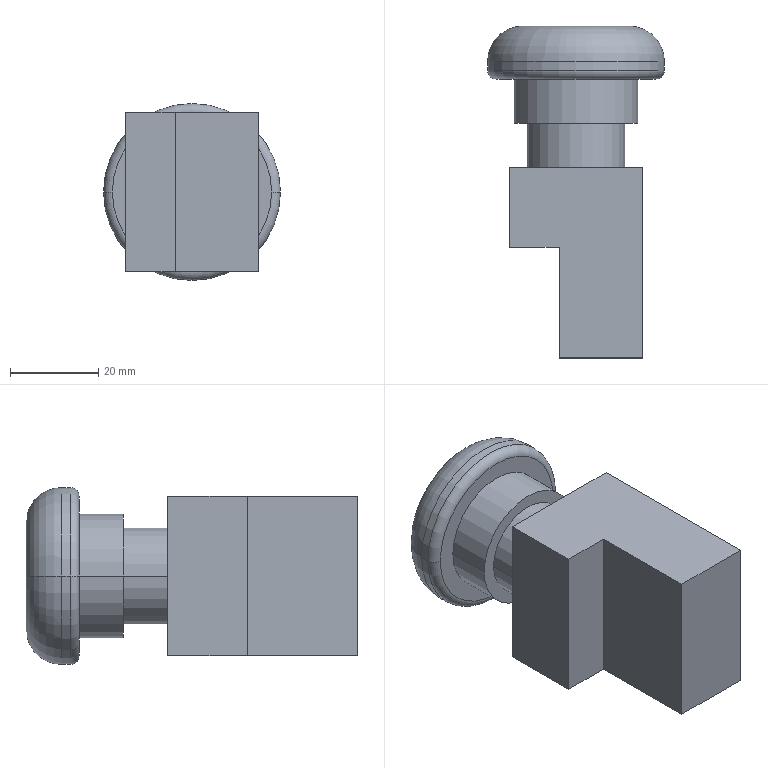Component | SolidWorks | EmergencyStopSwitch122-1 | 1 solid | 21 faces | box 40 x 75 x 40 mm | volume 59732 mm3 | plane 11 | cylinder 6 | torus 4 | commonest cylinder face diameters 22 x2 28 x2 40 x2
build123d program:
from build123d import *

# Parameters (mm, degrees)
EXTRUDE1_DEPTH      = 18
EXTRUDE1_DEPTH_BACK = 18
FILLET1_R           = 8
FILLET2_R           = 2


with BuildPart() as part:
    # Sketch1 → Extrude1 (new, two sides: drawn at the far end of the back side and taken through both)
    with BuildSketch(Plane.XY.offset(-EXTRUDE1_DEPTH_BACK)):
        Polygon((0, 0), (30, 0), (30, 18), (18.812, 18), (18.812, 43), (0, 43), align=None)
    extrude(amount=EXTRUDE1_DEPTH + EXTRUDE1_DEPTH_BACK)

    # Sketch2 → Revolve1 (revolve)
    with BuildSketch(Plane.XY, mode=Mode.PRIVATE) as revolve1_sk:
        Polygon((26, 0), (26, -10), (29, -10), (29, -20), (35, -20), (35, -32), (15, -32), (15, 0), align=None)
    revolve(revolve1_sk.sketch.rotate(Axis((15, 0, 0), (0, -1, 0)), 180), axis=Axis((15, 0, 0), (0, -1, 0)))

    # Fillet1
    fillet1_edges = [part.edges().sort_by_distance(p)[0] for p in [
        (35, -32, 0),
    ]]
    fillet(fillet1_edges, radius=FILLET1_R)

    # Fillet2
    fillet2_edges = [part.edges().sort_by_distance(p)[0] for p in [
        (35, -20, 0),
    ]]
    fillet(fillet2_edges, radius=FILLET2_R)


solid = part.part

# Placed as in the assembly
solid = solid.moved(Location((-497.479, 564.741, 730), (0, 0, 180)))
STEP:
#1=COLOUR_RGB('',0.7922,0.8196,0.9333);
#2=FILL_AREA_STYLE_COLOUR('',#1);
#3=FILL_AREA_STYLE('',(#2));
#4=SURFACE_STYLE_FILL_AREA(#3);
#5=SURFACE_SIDE_STYLE('',(#4));
#6=SURFACE_STYLE_USAGE(.BOTH.,#5);
#7=PRESENTATION_STYLE_ASSIGNMENT((#6));
#8=CARTESIAN_POINT('',(-19.468,23.021,28.74));
#9=VERTEX_POINT('',#8);
#10=CARTESIAN_POINT('',(-20.885,23.021,28.74));
#11=VERTEX_POINT('',#10);
#12=CARTESIAN_POINT('',(-20.176,23.021,28.74));
#13=DIRECTION('',(-0.,-1.,-0.));
#14=DIRECTION('',(-1.,0.,0.));
#15=AXIS2_PLACEMENT_3D('',#12,#13,#14);
#16=CIRCLE('',#15,0.7087);
#17=EDGE_CURVE('',#9,#11,#16,.T.);
#18=ORIENTED_EDGE('',*,*,#17,.F.);
#19=CARTESIAN_POINT('',(-19.389,23.1,28.74));
#20=VERTEX_POINT('',#19);
#21=CARTESIAN_POINT('',(-19.468,23.1,28.74));
#22=DIRECTION('',(-0.,0.,1.));
#23=DIRECTION('',(1.,0.,0.));
#24=AXIS2_PLACEMENT_3D('',#21,#22,#23);
#25=CIRCLE('',#24,0.07874);
#26=EDGE_CURVE('',#9,#20,#25,.T.);
#27=ORIENTED_EDGE('',*,*,#26,.T.);
#28=CARTESIAN_POINT('',(-20.964,23.1,28.74));
#29=VERTEX_POINT('',#28);
#30=CARTESIAN_POINT('',(-20.176,23.1,28.74));
#31=DIRECTION('',(0.,1.,0.));
#32=DIRECTION('',(-1.,0.,0.));
#33=AXIS2_PLACEMENT_3D('',#30,#31,#32);
#34=CIRCLE('',#33,0.7874);
#35=EDGE_CURVE('',#29,#20,#34,.T.);
#36=ORIENTED_EDGE('',*,*,#35,.F.);
#37=CARTESIAN_POINT('',(-20.885,23.1,28.74));
#38=DIRECTION('',(0.,0.,-1.));
#39=DIRECTION('',(0.,1.,0.));
#40=AXIS2_PLACEMENT_3D('',#37,#38,#39);
#41=CIRCLE('',#40,0.07874);
#42=EDGE_CURVE('',#11,#29,#41,.T.);
#43=ORIENTED_EDGE('',*,*,#42,.F.);
#44=EDGE_LOOP('',(#18,#27,#36,#43));
#45=FACE_OUTER_BOUND('',#44,.T.);
#46=CARTESIAN_POINT('',(-20.176,23.1,28.74));
#47=DIRECTION('',(0.,1.,0.));
#48=DIRECTION('',(-1.,0.,0.));
#49=AXIS2_PLACEMENT_3D('',#46,#47,#48);
#50=TOROIDAL_SURFACE('',#49,0.7087,0.07874);
#51=ADVANCED_FACE('',(#45),#50,.T.);
#52=CARTESIAN_POINT('',(-20.649,23.494,28.74));
#53=VERTEX_POINT('',#52);
#54=CARTESIAN_POINT('',(-19.704,23.494,28.74));
#55=VERTEX_POINT('',#54);
#56=CARTESIAN_POINT('',(-20.176,23.494,28.74));
#57=DIRECTION('',(0.,1.,0.));
#58=DIRECTION('',(1.,0.,0.));
#59=AXIS2_PLACEMENT_3D('',#56,#57,#58);
#60=CIRCLE('',#59,0.4724);
#61=EDGE_CURVE('',#53,#55,#60,.T.);
#62=ORIENTED_EDGE('',*,*,#61,.F.);
#63=CARTESIAN_POINT('',(-20.964,23.179,28.74));
#64=VERTEX_POINT('',#63);
#65=CARTESIAN_POINT('',(-20.649,23.179,28.74));
#66=DIRECTION('',(0.,-0.,1.));
#67=DIRECTION('',(1.,0.,0.));
#68=AXIS2_PLACEMENT_3D('',#65,#66,#67);
#69=CIRCLE('',#68,0.315);
#70=EDGE_CURVE('',#53,#64,#69,.T.);
#71=ORIENTED_EDGE('',*,*,#70,.T.);
#72=CARTESIAN_POINT('',(-19.389,23.179,28.74));
#73=VERTEX_POINT('',#72);
#74=CARTESIAN_POINT('',(-20.176,23.179,28.74));
#75=DIRECTION('',(-0.,-1.,-0.));
#76=DIRECTION('',(1.,0.,0.));
#77=AXIS2_PLACEMENT_3D('',#74,#75,#76);
#78=CIRCLE('',#77,0.7874);
#79=EDGE_CURVE('',#73,#64,#78,.T.);
#80=ORIENTED_EDGE('',*,*,#79,.F.);
#81=CARTESIAN_POINT('',(-19.704,23.179,28.74));
#82=DIRECTION('',(0.,0.,-1.));
#83=DIRECTION('',(0.,1.,0.));
#84=AXIS2_PLACEMENT_3D('',#81,#82,#83);
#85=CIRCLE('',#84,0.315);
#86=EDGE_CURVE('',#55,#73,#85,.T.);
#87=ORIENTED_EDGE('',*,*,#86,.F.);
#88=EDGE_LOOP('',(#62,#71,#80,#87));
#89=FACE_OUTER_BOUND('',#88,.T.);
#90=CARTESIAN_POINT('',(-20.176,23.179,28.74));
#91=DIRECTION('',(-0.,-1.,-0.));
#92=DIRECTION('',(1.,-0.,-0.));
#93=AXIS2_PLACEMENT_3D('',#90,#91,#92);
#94=TOROIDAL_SURFACE('',#93,0.4724,0.315);
#95=ADVANCED_FACE('',(#89),#94,.T.);
#96=CARTESIAN_POINT('',(-19.743,22.628,28.74));
#97=VERTEX_POINT('',#96);
#98=CARTESIAN_POINT('',(-20.609,22.628,28.74));
#99=VERTEX_POINT('',#98);
#100=CARTESIAN_POINT('',(-20.176,22.628,28.74));
#101=DIRECTION('',(-0.,-1.,-0.));
#102=DIRECTION('',(1.,0.,0.));
#103=AXIS2_PLACEMENT_3D('',#100,#101,#102);
#104=CIRCLE('',#103,0.4331);
#105=EDGE_CURVE('',#97,#99,#104,.T.);
#106=ORIENTED_EDGE('',*,*,#105,.T.);
#107=CARTESIAN_POINT('',(-20.609,22.234,28.74));
#108=VERTEX_POINT('',#107);
#109=CARTESIAN_POINT('',(-20.609,22.234,28.74));
#110=DIRECTION('',(-0.,-1.,-0.));
#111=VECTOR('',#110,39.37);
#112=LINE('',#109,#111);
#113=EDGE_CURVE('',#99,#108,#112,.T.);
#114=ORIENTED_EDGE('',*,*,#113,.T.);
#115=CARTESIAN_POINT('',(-19.743,22.234,28.74));
#116=VERTEX_POINT('',#115);
#117=CARTESIAN_POINT('',(-20.176,22.234,28.74));
#118=DIRECTION('',(0.,1.,0.));
#119=DIRECTION('',(0.,0.,1.));
#120=AXIS2_PLACEMENT_3D('',#117,#118,#119);
#121=CIRCLE('',#120,0.4331);
#122=EDGE_CURVE('',#108,#116,#121,.T.);
#123=ORIENTED_EDGE('',*,*,#122,.T.);
#124=CARTESIAN_POINT('',(-19.743,22.234,28.74));
#125=DIRECTION('',(-0.,-1.,-0.));
#126=VECTOR('',#125,39.37);
#127=LINE('',#124,#126);
#128=EDGE_CURVE('',#97,#116,#127,.T.);
#129=ORIENTED_EDGE('',*,*,#128,.F.);
#130=EDGE_LOOP('',(#106,#114,#123,#129));
#131=FACE_OUTER_BOUND('',#130,.T.);
#132=CARTESIAN_POINT('',(-20.176,22.234,28.74));
#133=DIRECTION('',(-0.,-1.,-0.));
#134=DIRECTION('',(1.,0.,0.));
#135=AXIS2_PLACEMENT_3D('',#132,#133,#134);
#136=CYLINDRICAL_SURFACE('',#135,0.4331);
#137=ADVANCED_FACE('',(#131),#136,.T.);
#138=CARTESIAN_POINT('',(-19.625,23.021,28.74));
#139=VERTEX_POINT('',#138);
#140=CARTESIAN_POINT('',(-20.728,23.021,28.74));
#141=VERTEX_POINT('',#140);
#142=CARTESIAN_POINT('',(-20.176,23.021,28.74));
#143=DIRECTION('',(-0.,-1.,-0.));
#144=DIRECTION('',(1.,0.,0.));
#145=AXIS2_PLACEMENT_3D('',#142,#143,#144);
#146=CIRCLE('',#145,0.5512);
#147=EDGE_CURVE('',#139,#141,#146,.T.);
#148=ORIENTED_EDGE('',*,*,#147,.T.);
#149=CARTESIAN_POINT('',(-20.728,22.628,28.74));
#150=VERTEX_POINT('',#149);
#151=CARTESIAN_POINT('',(-20.728,22.234,28.74));
#152=DIRECTION('',(-0.,-1.,-0.));
#153=VECTOR('',#152,39.37);
#154=LINE('',#151,#153);
#155=EDGE_CURVE('',#141,#150,#154,.T.);
#156=ORIENTED_EDGE('',*,*,#155,.T.);
#157=CARTESIAN_POINT('',(-19.625,22.628,28.74));
#158=VERTEX_POINT('',#157);
#159=CARTESIAN_POINT('',(-20.176,22.628,28.74));
#160=DIRECTION('',(-0.,-1.,-0.));
#161=DIRECTION('',(1.,0.,0.));
#162=AXIS2_PLACEMENT_3D('',#159,#160,#161);
#163=CIRCLE('',#162,0.5512);
#164=EDGE_CURVE('',#158,#150,#163,.T.);
#165=ORIENTED_EDGE('',*,*,#164,.F.);
#166=CARTESIAN_POINT('',(-19.625,22.234,28.74));
#167=DIRECTION('',(-0.,-1.,-0.));
#168=VECTOR('',#167,39.37);
#169=LINE('',#166,#168);
#170=EDGE_CURVE('',#139,#158,#169,.T.);
#171=ORIENTED_EDGE('',*,*,#170,.F.);
#172=EDGE_LOOP('',(#148,#156,#165,#171));
#173=FACE_OUTER_BOUND('',#172,.T.);
#174=CARTESIAN_POINT('',(-20.176,22.234,28.74));
#175=DIRECTION('',(-0.,-1.,-0.));
#176=DIRECTION('',(1.,0.,0.));
#177=AXIS2_PLACEMENT_3D('',#174,#175,#176);
#178=CYLINDRICAL_SURFACE('',#177,0.5512);
#179=ADVANCED_FACE('',(#173),#178,.T.);
#180=ORIENTED_EDGE('',*,*,#79,.T.);
#181=CARTESIAN_POINT('',(-20.964,22.234,28.74));
#182=DIRECTION('',(-0.,-1.,-0.));
#183=VECTOR('',#182,39.37);
#184=LINE('',#181,#183);
#185=EDGE_CURVE('',#64,#29,#184,.T.);
#186=ORIENTED_EDGE('',*,*,#185,.T.);
#187=ORIENTED_EDGE('',*,*,#35,.T.);
#188=CARTESIAN_POINT('',(-19.389,22.234,28.74));
#189=DIRECTION('',(-0.,-1.,-0.));
#190=VECTOR('',#189,39.37);
#191=LINE('',#188,#190);
#192=EDGE_CURVE('',#73,#20,#191,.T.);
#193=ORIENTED_EDGE('',*,*,#192,.F.);
#194=EDGE_LOOP('',(#180,#186,#187,#193));
#195=FACE_OUTER_BOUND('',#194,.T.);
#196=CARTESIAN_POINT('',(-20.176,22.234,28.74));
#197=DIRECTION('',(-0.,-1.,-0.));
#198=DIRECTION('',(1.,0.,0.));
#199=AXIS2_PLACEMENT_3D('',#196,#197,#198);
#200=CYLINDRICAL_SURFACE('',#199,0.7874);
#201=ADVANCED_FACE('',(#195),#200,.T.);
#202=CARTESIAN_POINT('',(-19.586,22.234,29.449));
#203=VERTEX_POINT('',#202);
#204=CARTESIAN_POINT('',(-19.586,22.234,28.031));
#205=VERTEX_POINT('',#204);
#206=CARTESIAN_POINT('',(-19.586,22.234,29.449));
#207=DIRECTION('',(0.,0.,-1.));
#208=VECTOR('',#207,39.37);
#209=LINE('',#206,#208);
#210=EDGE_CURVE('',#203,#205,#209,.T.);
#211=ORIENTED_EDGE('',*,*,#210,.T.);
#212=CARTESIAN_POINT('',(-20.767,22.234,28.031));
#213=VERTEX_POINT('',#212);
#214=CARTESIAN_POINT('',(-19.586,22.234,28.031));
#215=DIRECTION('',(-1.,0.,0.));
#216=VECTOR('',#215,39.37);
#217=LINE('',#214,#216);
#218=EDGE_CURVE('',#205,#213,#217,.T.);
#219=ORIENTED_EDGE('',*,*,#218,.T.);
#220=CARTESIAN_POINT('',(-20.767,22.234,29.449));
#221=VERTEX_POINT('',#220);
#222=CARTESIAN_POINT('',(-20.767,22.234,29.449));
#223=DIRECTION('',(0.,0.,-1.));
#224=VECTOR('',#223,39.37);
#225=LINE('',#222,#224);
#226=EDGE_CURVE('',#221,#213,#225,.T.);
#227=ORIENTED_EDGE('',*,*,#226,.F.);
#228=CARTESIAN_POINT('',(-19.586,22.234,29.449));
#229=DIRECTION('',(-1.,0.,0.));
#230=VECTOR('',#229,39.37);
#231=LINE('',#228,#230);
#232=EDGE_CURVE('',#203,#221,#231,.T.);
#233=ORIENTED_EDGE('',*,*,#232,.F.);
#234=EDGE_LOOP('',(#211,#219,#227,#233));
#235=FACE_OUTER_BOUND('',#234,.T.);
#236=CARTESIAN_POINT('',(-20.176,22.234,28.74));
#237=DIRECTION('',(0.,1.,0.));
#238=DIRECTION('',(0.,0.,1.));
#239=AXIS2_PLACEMENT_3D('',#236,#237,#238);
#240=CIRCLE('',#239,0.4331);
#241=EDGE_CURVE('',#116,#108,#240,.T.);
#242=ORIENTED_EDGE('',*,*,#241,.F.);
#243=ORIENTED_EDGE('',*,*,#122,.F.);
#244=EDGE_LOOP('',(#242,#243));
#245=FACE_BOUND('',#244,.T.);
#246=CARTESIAN_POINT('',(-19.586,22.234,29.449));
#247=DIRECTION('',(-0.,-1.,-0.));
#248=DIRECTION('',(-0.,-0.,1.));
#249=AXIS2_PLACEMENT_3D('',#246,#247,#248);
#250=PLANE('',#249);
#251=ADVANCED_FACE('',(#235,#245),#250,.F.);
#252=CARTESIAN_POINT('',(-19.586,20.541,29.449));
#253=VERTEX_POINT('',#252);
#254=CARTESIAN_POINT('',(-19.586,20.541,28.031));
#255=VERTEX_POINT('',#254);
#256=CARTESIAN_POINT('',(-19.586,20.541,29.449));
#257=DIRECTION('',(0.,0.,-1.));
#258=VECTOR('',#257,39.37);
#259=LINE('',#256,#258);
#260=EDGE_CURVE('',#253,#255,#259,.T.);
#261=ORIENTED_EDGE('',*,*,#260,.T.);
#262=CARTESIAN_POINT('',(-19.586,22.234,28.031));
#263=DIRECTION('',(0.,1.,0.));
#264=VECTOR('',#263,39.37);
#265=LINE('',#262,#264);
#266=EDGE_CURVE('',#255,#205,#265,.T.);
#267=ORIENTED_EDGE('',*,*,#266,.T.);
#268=ORIENTED_EDGE('',*,*,#210,.F.);
#269=CARTESIAN_POINT('',(-19.586,22.234,29.449));
#270=DIRECTION('',(0.,1.,0.));
#271=VECTOR('',#270,39.37);
#272=LINE('',#269,#271);
#273=EDGE_CURVE('',#253,#203,#272,.T.);
#274=ORIENTED_EDGE('',*,*,#273,.F.);
#275=EDGE_LOOP('',(#261,#267,#268,#274));
#276=FACE_OUTER_BOUND('',#275,.T.);
#277=CARTESIAN_POINT('',(-19.586,22.234,29.449));
#278=DIRECTION('',(-1.,0.,0.));
#279=DIRECTION('',(0.,0.,-1.));
#280=AXIS2_PLACEMENT_3D('',#277,#278,#279);
#281=PLANE('',#280);
#282=ADVANCED_FACE('',(#276),#281,.F.);
#283=ORIENTED_EDGE('',*,*,#226,.T.);
#284=CARTESIAN_POINT('',(-20.767,21.525,28.031));
#285=VERTEX_POINT('',#284);
#286=CARTESIAN_POINT('',(-20.767,22.234,28.031));
#287=DIRECTION('',(-0.,-1.,-0.));
#288=VECTOR('',#287,39.37);
#289=LINE('',#286,#288);
#290=EDGE_CURVE('',#213,#285,#289,.T.);
#291=ORIENTED_EDGE('',*,*,#290,.T.);
#292=CARTESIAN_POINT('',(-20.767,21.525,29.449));
#293=VERTEX_POINT('',#292);
#294=CARTESIAN_POINT('',(-20.767,21.525,29.449));
#295=DIRECTION('',(0.,0.,-1.));
#296=VECTOR('',#295,39.37);
#297=LINE('',#294,#296);
#298=EDGE_CURVE('',#293,#285,#297,.T.);
#299=ORIENTED_EDGE('',*,*,#298,.F.);
#300=CARTESIAN_POINT('',(-20.767,22.234,29.449));
#301=DIRECTION('',(-0.,-1.,-0.));
#302=VECTOR('',#301,39.37);
#303=LINE('',#300,#302);
#304=EDGE_CURVE('',#221,#293,#303,.T.);
#305=ORIENTED_EDGE('',*,*,#304,.F.);
#306=EDGE_LOOP('',(#283,#291,#299,#305));
#307=FACE_OUTER_BOUND('',#306,.T.);
#308=CARTESIAN_POINT('',(-20.767,22.234,29.449));
#309=DIRECTION('',(1.,-0.,0.));
#310=DIRECTION('',(-0.,-0.,1.));
#311=AXIS2_PLACEMENT_3D('',#308,#309,#310);
#312=PLANE('',#311);
#313=ADVANCED_FACE('',(#307),#312,.F.);
#314=ORIENTED_EDGE('',*,*,#298,.T.);
#315=CARTESIAN_POINT('',(-20.326,21.525,28.031));
#316=VERTEX_POINT('',#315);
#317=CARTESIAN_POINT('',(-20.767,21.525,28.031));
#318=DIRECTION('',(1.,-0.,0.));
#319=VECTOR('',#318,39.37);
#320=LINE('',#317,#319);
#321=EDGE_CURVE('',#285,#316,#320,.T.);
#322=ORIENTED_EDGE('',*,*,#321,.T.);
#323=CARTESIAN_POINT('',(-20.326,21.525,29.449));
#324=VERTEX_POINT('',#323);
#325=CARTESIAN_POINT('',(-20.326,21.525,29.449));
#326=DIRECTION('',(0.,0.,-1.));
#327=VECTOR('',#326,39.37);
#328=LINE('',#325,#327);
#329=EDGE_CURVE('',#324,#316,#328,.T.);
#330=ORIENTED_EDGE('',*,*,#329,.F.);
#331=CARTESIAN_POINT('',(-20.767,21.525,29.449));
#332=DIRECTION('',(1.,-0.,0.));
#333=VECTOR('',#332,39.37);
#334=LINE('',#331,#333);
#335=EDGE_CURVE('',#293,#324,#334,.T.);
#336=ORIENTED_EDGE('',*,*,#335,.F.);
#337=EDGE_LOOP('',(#314,#322,#330,#336));
#338=FACE_OUTER_BOUND('',#337,.T.);
#339=CARTESIAN_POINT('',(-20.767,21.525,29.449));
#340=DIRECTION('',(0.,1.,0.));
#341=DIRECTION('',(0.,0.,-1.));
#342=AXIS2_PLACEMENT_3D('',#339,#340,#341);
#343=PLANE('',#342);
#344=ADVANCED_FACE('',(#338),#343,.F.);
#345=ORIENTED_EDGE('',*,*,#329,.T.);
#346=CARTESIAN_POINT('',(-20.326,20.541,28.031));
#347=VERTEX_POINT('',#346);
#348=CARTESIAN_POINT('',(-20.326,20.541,28.031));
#349=DIRECTION('',(0.,-1.,-0.));
#350=VECTOR('',#349,39.37);
#351=LINE('',#348,#350);
#352=EDGE_CURVE('',#316,#347,#351,.T.);
#353=ORIENTED_EDGE('',*,*,#352,.T.);
#354=CARTESIAN_POINT('',(-20.326,20.541,29.449));
#355=VERTEX_POINT('',#354);
#356=CARTESIAN_POINT('',(-20.326,20.541,29.449));
#357=DIRECTION('',(0.,0.,-1.));
#358=VECTOR('',#357,39.37);
#359=LINE('',#356,#358);
#360=EDGE_CURVE('',#355,#347,#359,.T.);
#361=ORIENTED_EDGE('',*,*,#360,.F.);
#362=CARTESIAN_POINT('',(-20.326,20.541,29.449));
#363=DIRECTION('',(0.,-1.,-0.));
#364=VECTOR('',#363,39.37);
#365=LINE('',#362,#364);
#366=EDGE_CURVE('',#324,#355,#365,.T.);
#367=ORIENTED_EDGE('',*,*,#366,.F.);
#368=EDGE_LOOP('',(#345,#353,#361,#367));
#369=FACE_OUTER_BOUND('',#368,.T.);
#370=CARTESIAN_POINT('',(-20.326,20.541,29.449));
#371=DIRECTION('',(1.,0.,0.));
#372=DIRECTION('',(-0.,1.,0.));
#373=AXIS2_PLACEMENT_3D('',#370,#371,#372);
#374=PLANE('',#373);
#375=ADVANCED_FACE('',(#369),#374,.F.);
#376=ORIENTED_EDGE('',*,*,#360,.T.);
#377=CARTESIAN_POINT('',(-19.586,20.541,28.031));
#378=DIRECTION('',(1.,-0.,0.));
#379=VECTOR('',#378,39.37);
#380=LINE('',#377,#379);
#381=EDGE_CURVE('',#347,#255,#380,.T.);
#382=ORIENTED_EDGE('',*,*,#381,.T.);
#383=ORIENTED_EDGE('',*,*,#260,.F.);
#384=CARTESIAN_POINT('',(-19.586,20.541,29.449));
#385=DIRECTION('',(1.,-0.,0.));
#386=VECTOR('',#385,39.37);
#387=LINE('',#384,#386);
#388=EDGE_CURVE('',#355,#253,#387,.T.);
#389=ORIENTED_EDGE('',*,*,#388,.F.);
#390=EDGE_LOOP('',(#376,#382,#383,#389));
#391=FACE_OUTER_BOUND('',#390,.T.);
#392=CARTESIAN_POINT('',(-19.586,20.541,29.449));
#393=DIRECTION('',(0.,1.,0.));
#394=DIRECTION('',(0.,0.,-1.));
#395=AXIS2_PLACEMENT_3D('',#392,#393,#394);
#396=PLANE('',#395);
#397=ADVANCED_FACE('',(#391),#396,.F.);
#398=ORIENTED_EDGE('',*,*,#273,.T.);
#399=ORIENTED_EDGE('',*,*,#232,.T.);
#400=ORIENTED_EDGE('',*,*,#304,.T.);
#401=ORIENTED_EDGE('',*,*,#335,.T.);
#402=ORIENTED_EDGE('',*,*,#366,.T.);
#403=ORIENTED_EDGE('',*,*,#388,.T.);
#404=EDGE_LOOP('',(#398,#399,#400,#401,#402,#403));
#405=FACE_OUTER_BOUND('',#404,.T.);
#406=CARTESIAN_POINT('',(-19.586,20.541,29.449));
#407=DIRECTION('',(0.,0.,-1.));
#408=DIRECTION('',(1.,-0.,0.));
#409=AXIS2_PLACEMENT_3D('',#406,#407,#408);
#410=PLANE('',#409);
#411=ADVANCED_FACE('',(#405),#410,.F.);
#412=ORIENTED_EDGE('',*,*,#266,.F.);
#413=ORIENTED_EDGE('',*,*,#381,.F.);
#414=ORIENTED_EDGE('',*,*,#352,.F.);
#415=ORIENTED_EDGE('',*,*,#321,.F.);
#416=ORIENTED_EDGE('',*,*,#290,.F.);
#417=ORIENTED_EDGE('',*,*,#218,.F.);
#418=EDGE_LOOP('',(#412,#413,#414,#415,#416,#417));
#419=FACE_OUTER_BOUND('',#418,.T.);
#420=CARTESIAN_POINT('',(-19.586,20.541,28.031));
#421=DIRECTION('',(0.,0.,-1.));
#422=DIRECTION('',(1.,-0.,0.));
#423=AXIS2_PLACEMENT_3D('',#420,#421,#422);
#424=PLANE('',#423);
#425=ADVANCED_FACE('',(#419),#424,.T.);
#426=CARTESIAN_POINT('',(-20.176,23.494,28.74));
#427=DIRECTION('',(0.,1.,0.));
#428=DIRECTION('',(1.,0.,0.));
#429=AXIS2_PLACEMENT_3D('',#426,#427,#428);
#430=CIRCLE('',#429,0.4724);
#431=EDGE_CURVE('',#55,#53,#430,.T.);
#432=ORIENTED_EDGE('',*,*,#431,.T.);
#433=ORIENTED_EDGE('',*,*,#61,.T.);
#434=EDGE_LOOP('',(#432,#433));
#435=FACE_OUTER_BOUND('',#434,.T.);
#436=CARTESIAN_POINT('',(-20.176,23.494,28.74));
#437=DIRECTION('',(-0.,-1.,-0.));
#438=DIRECTION('',(1.,-0.,-0.));
#439=AXIS2_PLACEMENT_3D('',#436,#437,#438);
#440=PLANE('',#439);
#441=ADVANCED_FACE('',(#435),#440,.F.);
#442=ORIENTED_EDGE('',*,*,#185,.F.);
#443=CARTESIAN_POINT('',(-20.176,23.179,28.74));
#444=DIRECTION('',(-0.,-1.,-0.));
#445=DIRECTION('',(1.,0.,0.));
#446=AXIS2_PLACEMENT_3D('',#443,#444,#445);
#447=CIRCLE('',#446,0.7874);
#448=EDGE_CURVE('',#64,#73,#447,.T.);
#449=ORIENTED_EDGE('',*,*,#448,.T.);
#450=ORIENTED_EDGE('',*,*,#192,.T.);
#451=CARTESIAN_POINT('',(-20.176,23.1,28.74));
#452=DIRECTION('',(0.,1.,0.));
#453=DIRECTION('',(-1.,0.,0.));
#454=AXIS2_PLACEMENT_3D('',#451,#452,#453);
#455=CIRCLE('',#454,0.7874);
#456=EDGE_CURVE('',#20,#29,#455,.T.);
#457=ORIENTED_EDGE('',*,*,#456,.T.);
#458=EDGE_LOOP('',(#442,#449,#450,#457));
#459=FACE_OUTER_BOUND('',#458,.T.);
#460=CARTESIAN_POINT('',(-20.176,22.234,28.74));
#461=DIRECTION('',(-0.,-1.,-0.));
#462=DIRECTION('',(1.,0.,0.));
#463=AXIS2_PLACEMENT_3D('',#460,#461,#462);
#464=CYLINDRICAL_SURFACE('',#463,0.7874);
#465=ADVANCED_FACE('',(#459),#464,.T.);
#466=CARTESIAN_POINT('',(-20.176,23.021,28.74));
#467=DIRECTION('',(-0.,-1.,-0.));
#468=DIRECTION('',(-1.,0.,0.));
#469=AXIS2_PLACEMENT_3D('',#466,#467,#468);
#470=CIRCLE('',#469,0.7087);
#471=EDGE_CURVE('',#11,#9,#470,.T.);
#472=ORIENTED_EDGE('',*,*,#471,.T.);
#473=ORIENTED_EDGE('',*,*,#17,.T.);
#474=EDGE_LOOP('',(#472,#473));
#475=FACE_OUTER_BOUND('',#474,.T.);
#476=ORIENTED_EDGE('',*,*,#147,.F.);
#477=CARTESIAN_POINT('',(-20.176,23.021,28.74));
#478=DIRECTION('',(-0.,-1.,-0.));
#479=DIRECTION('',(1.,0.,0.));
#480=AXIS2_PLACEMENT_3D('',#477,#478,#479);
#481=CIRCLE('',#480,0.5512);
#482=EDGE_CURVE('',#141,#139,#481,.T.);
#483=ORIENTED_EDGE('',*,*,#482,.F.);
#484=EDGE_LOOP('',(#476,#483));
#485=FACE_BOUND('',#484,.T.);
#486=CARTESIAN_POINT('',(-20.728,23.021,28.74));
#487=DIRECTION('',(0.,1.,0.));
#488=DIRECTION('',(-1.,0.,0.));
#489=AXIS2_PLACEMENT_3D('',#486,#487,#488);
#490=PLANE('',#489);
#491=ADVANCED_FACE('',(#475,#485),#490,.F.);
#492=ORIENTED_EDGE('',*,*,#155,.F.);
#493=ORIENTED_EDGE('',*,*,#482,.T.);
#494=ORIENTED_EDGE('',*,*,#170,.T.);
#495=CARTESIAN_POINT('',(-20.176,22.628,28.74));
#496=DIRECTION('',(-0.,-1.,-0.));
#497=DIRECTION('',(1.,0.,0.));
#498=AXIS2_PLACEMENT_3D('',#495,#496,#497);
#499=CIRCLE('',#498,0.5512);
#500=EDGE_CURVE('',#150,#158,#499,.T.);
#501=ORIENTED_EDGE('',*,*,#500,.F.);
#502=EDGE_LOOP('',(#492,#493,#494,#501));
#503=FACE_OUTER_BOUND('',#502,.T.);
#504=CARTESIAN_POINT('',(-20.176,22.234,28.74));
#505=DIRECTION('',(-0.,-1.,-0.));
#506=DIRECTION('',(1.,0.,0.));
#507=AXIS2_PLACEMENT_3D('',#504,#505,#506);
#508=CYLINDRICAL_SURFACE('',#507,0.5512);
#509=ADVANCED_FACE('',(#503),#508,.T.);
#510=ORIENTED_EDGE('',*,*,#105,.F.);
#511=CARTESIAN_POINT('',(-20.176,22.628,28.74));
#512=DIRECTION('',(-0.,-1.,-0.));
#513=DIRECTION('',(1.,0.,0.));
#514=AXIS2_PLACEMENT_3D('',#511,#512,#513);
#515=CIRCLE('',#514,0.4331);
#516=EDGE_CURVE('',#99,#97,#515,.T.);
#517=ORIENTED_EDGE('',*,*,#516,.F.);
#518=EDGE_LOOP('',(#510,#517));
#519=FACE_BOUND('',#518,.T.);
#520=ORIENTED_EDGE('',*,*,#164,.T.);
#521=ORIENTED_EDGE('',*,*,#500,.T.);
#522=EDGE_LOOP('',(#520,#521));
#523=FACE_OUTER_BOUND('',#522,.T.);
#524=CARTESIAN_POINT('',(-20.609,22.628,28.74));
#525=DIRECTION('',(0.,1.,0.));
#526=DIRECTION('',(-1.,0.,0.));
#527=AXIS2_PLACEMENT_3D('',#524,#525,#526);
#528=PLANE('',#527);
#529=ADVANCED_FACE('',(#519,#523),#528,.F.);
#530=ORIENTED_EDGE('',*,*,#113,.F.);
#531=ORIENTED_EDGE('',*,*,#516,.T.);
#532=ORIENTED_EDGE('',*,*,#128,.T.);
#533=ORIENTED_EDGE('',*,*,#241,.T.);
#534=EDGE_LOOP('',(#530,#531,#532,#533));
#535=FACE_OUTER_BOUND('',#534,.T.);
#536=CARTESIAN_POINT('',(-20.176,22.234,28.74));
#537=DIRECTION('',(-0.,-1.,-0.));
#538=DIRECTION('',(1.,0.,0.));
#539=AXIS2_PLACEMENT_3D('',#536,#537,#538);
#540=CYLINDRICAL_SURFACE('',#539,0.4331);
#541=ADVANCED_FACE('',(#535),#540,.T.);
#542=ORIENTED_EDGE('',*,*,#70,.F.);
#543=ORIENTED_EDGE('',*,*,#431,.F.);
#544=ORIENTED_EDGE('',*,*,#86,.T.);
#545=ORIENTED_EDGE('',*,*,#448,.F.);
#546=EDGE_LOOP('',(#542,#543,#544,#545));
#547=FACE_OUTER_BOUND('',#546,.T.);
#548=CARTESIAN_POINT('',(-20.176,23.179,28.74));
#549=DIRECTION('',(-0.,-1.,-0.));
#550=DIRECTION('',(1.,-0.,-0.));
#551=AXIS2_PLACEMENT_3D('',#548,#549,#550);
#552=TOROIDAL_SURFACE('',#551,0.4724,0.315);
#553=ADVANCED_FACE('',(#547),#552,.T.);
#554=ORIENTED_EDGE('',*,*,#26,.F.);
#555=ORIENTED_EDGE('',*,*,#471,.F.);
#556=ORIENTED_EDGE('',*,*,#42,.T.);
#557=ORIENTED_EDGE('',*,*,#456,.F.);
#558=EDGE_LOOP('',(#554,#555,#556,#557));
#559=FACE_OUTER_BOUND('',#558,.T.);
#560=CARTESIAN_POINT('',(-20.176,23.1,28.74));
#561=DIRECTION('',(0.,1.,0.));
#562=DIRECTION('',(-1.,0.,0.));
#563=AXIS2_PLACEMENT_3D('',#560,#561,#562);
#564=TOROIDAL_SURFACE('',#563,0.7087,0.07874);
#565=ADVANCED_FACE('',(#559),#564,.T.);
#566=CLOSED_SHELL('',(#51,#95,#137,#179,#201,#251,#282,#313,#344,#375,#397,#411,#425,#441,#465,#491,#509,#529,#541,#553,#565));
#567=MANIFOLD_SOLID_BREP('',#566);
#568=STYLED_ITEM('',(#7),#567);
#569=(LENGTH_UNIT()NAMED_UNIT(*)SI_UNIT($,.METRE.));
#570=LENGTH_MEASURE_WITH_UNIT(LENGTH_MEASURE(0.0254),#569);
#571=DIMENSIONAL_EXPONENTS(1.,0.,0.,0.,0.,0.,0.);
#572=(CONVERSION_BASED_UNIT('',#570)LENGTH_UNIT()NAMED_UNIT(#571));
#573=UNCERTAINTY_MEASURE_WITH_UNIT(LENGTH_MEASURE(0.00001),#572,'','');
#574=(NAMED_UNIT(*)PLANE_ANGLE_UNIT()SI_UNIT($,.RADIAN.));
#575=(NAMED_UNIT(*)SI_UNIT($,.STERADIAN.)SOLID_ANGLE_UNIT());
#576=(GEOMETRIC_REPRESENTATION_CONTEXT(3)GLOBAL_UNCERTAINTY_ASSIGNED_CONTEXT((#573))GLOBAL_UNIT_ASSIGNED_CONTEXT((#572,#574,#575))REPRESENTATION_CONTEXT('',''));
#577=MECHANICAL_DESIGN_GEOMETRIC_PRESENTATION_REPRESENTATION('',(#568),#576);
#578=CARTESIAN_POINT('',(0.,0.,0.));
#579=DIRECTION('',(0.,0.,1.));
#580=DIRECTION('',(1.,0.,0.));
#581=AXIS2_PLACEMENT_3D('',#578,#579,#580);
#582=(LENGTH_UNIT()NAMED_UNIT(*)SI_UNIT($,.METRE.));
#583=LENGTH_MEASURE_WITH_UNIT(LENGTH_MEASURE(0.0254),#582);
#584=DIMENSIONAL_EXPONENTS(1.,0.,0.,0.,0.,0.,0.);
#585=(CONVERSION_BASED_UNIT('',#583)LENGTH_UNIT()NAMED_UNIT(#584));
#586=UNCERTAINTY_MEASURE_WITH_UNIT(LENGTH_MEASURE(0.00001),#585,'','');
#587=(NAMED_UNIT(*)PLANE_ANGLE_UNIT()SI_UNIT($,.RADIAN.));
#588=(NAMED_UNIT(*)SI_UNIT($,.STERADIAN.)SOLID_ANGLE_UNIT());
#589=(GEOMETRIC_REPRESENTATION_CONTEXT(3)GLOBAL_UNCERTAINTY_ASSIGNED_CONTEXT((#586))GLOBAL_UNIT_ASSIGNED_CONTEXT((#585,#587,#588))REPRESENTATION_CONTEXT('',''));
#590=ADVANCED_BREP_SHAPE_REPRESENTATION('',(#567,#581),#589);
#591=PRESENTATION_LAYER_ASSIGNMENT('','',(#568));